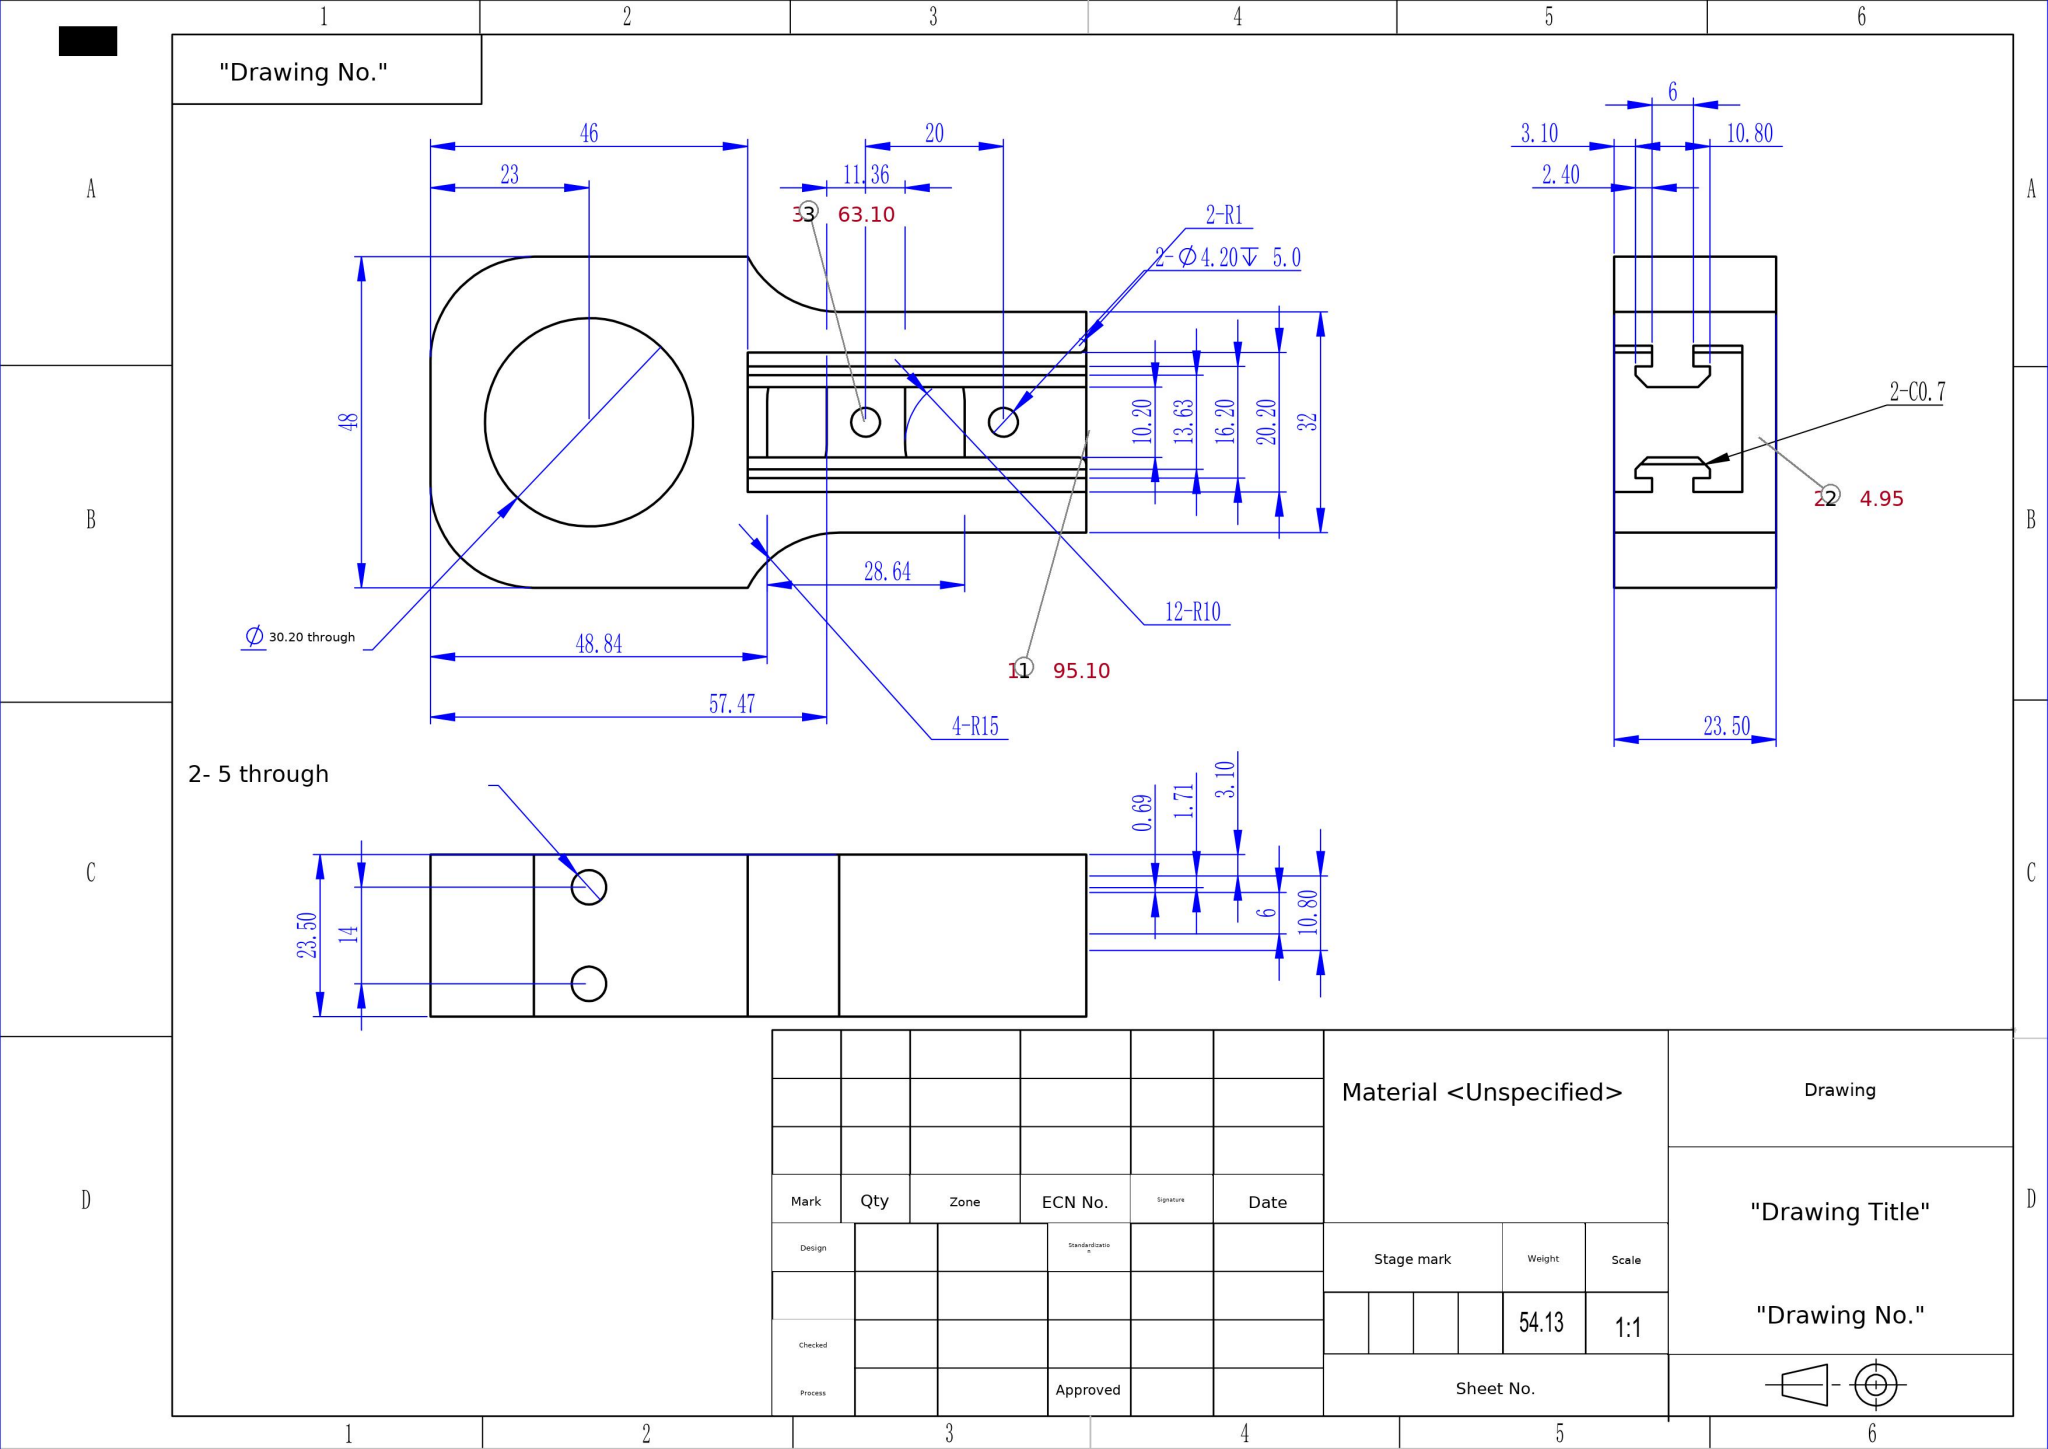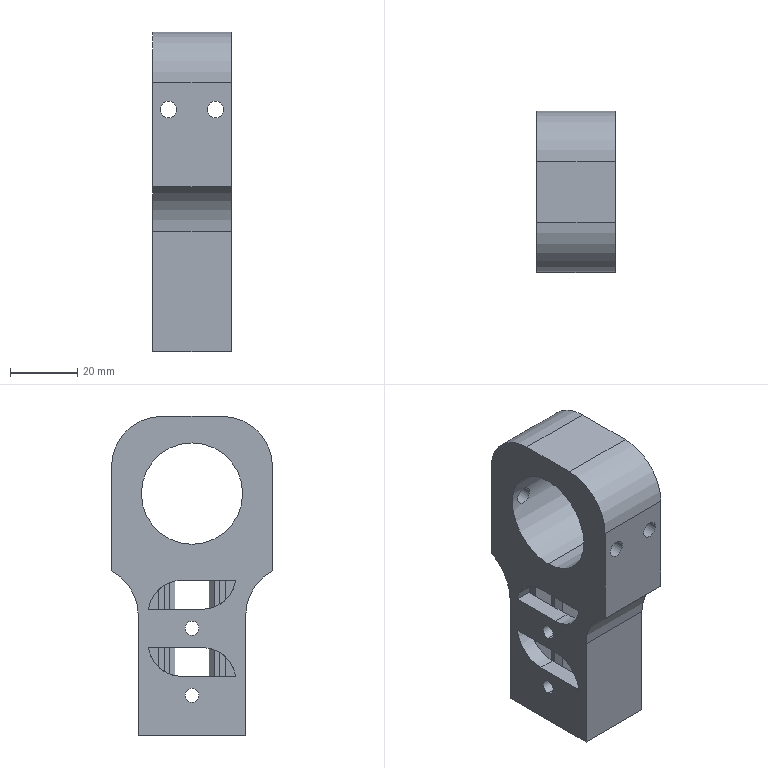Part | SolidWorks | mm | 1 solid | 67 faces | box 23.5 x 48 x 95.1 mm | volume 54126 mm3 | plane 42 | cylinder 25 | commonest cylinder face diameters 5 x8 4.2 x4 20 x4 30 x4 2 x3 30.2 x2